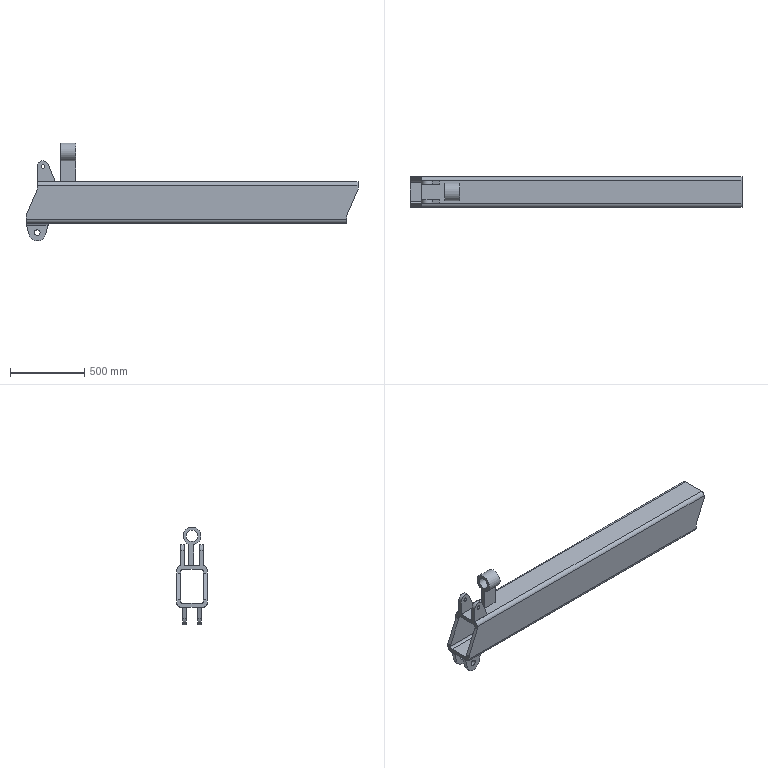Component | NX | ARM_SECTION_3 | 1 solid | 60 faces | volume 49024249 mm3 | plane 34 | cylinder 24 | spline 2 | commonest cylinder face diameters 30 x10 50 x4 114.3 x2 38.1 x2 76.2 x2 25.4 x2 120 x1 76.3 x1